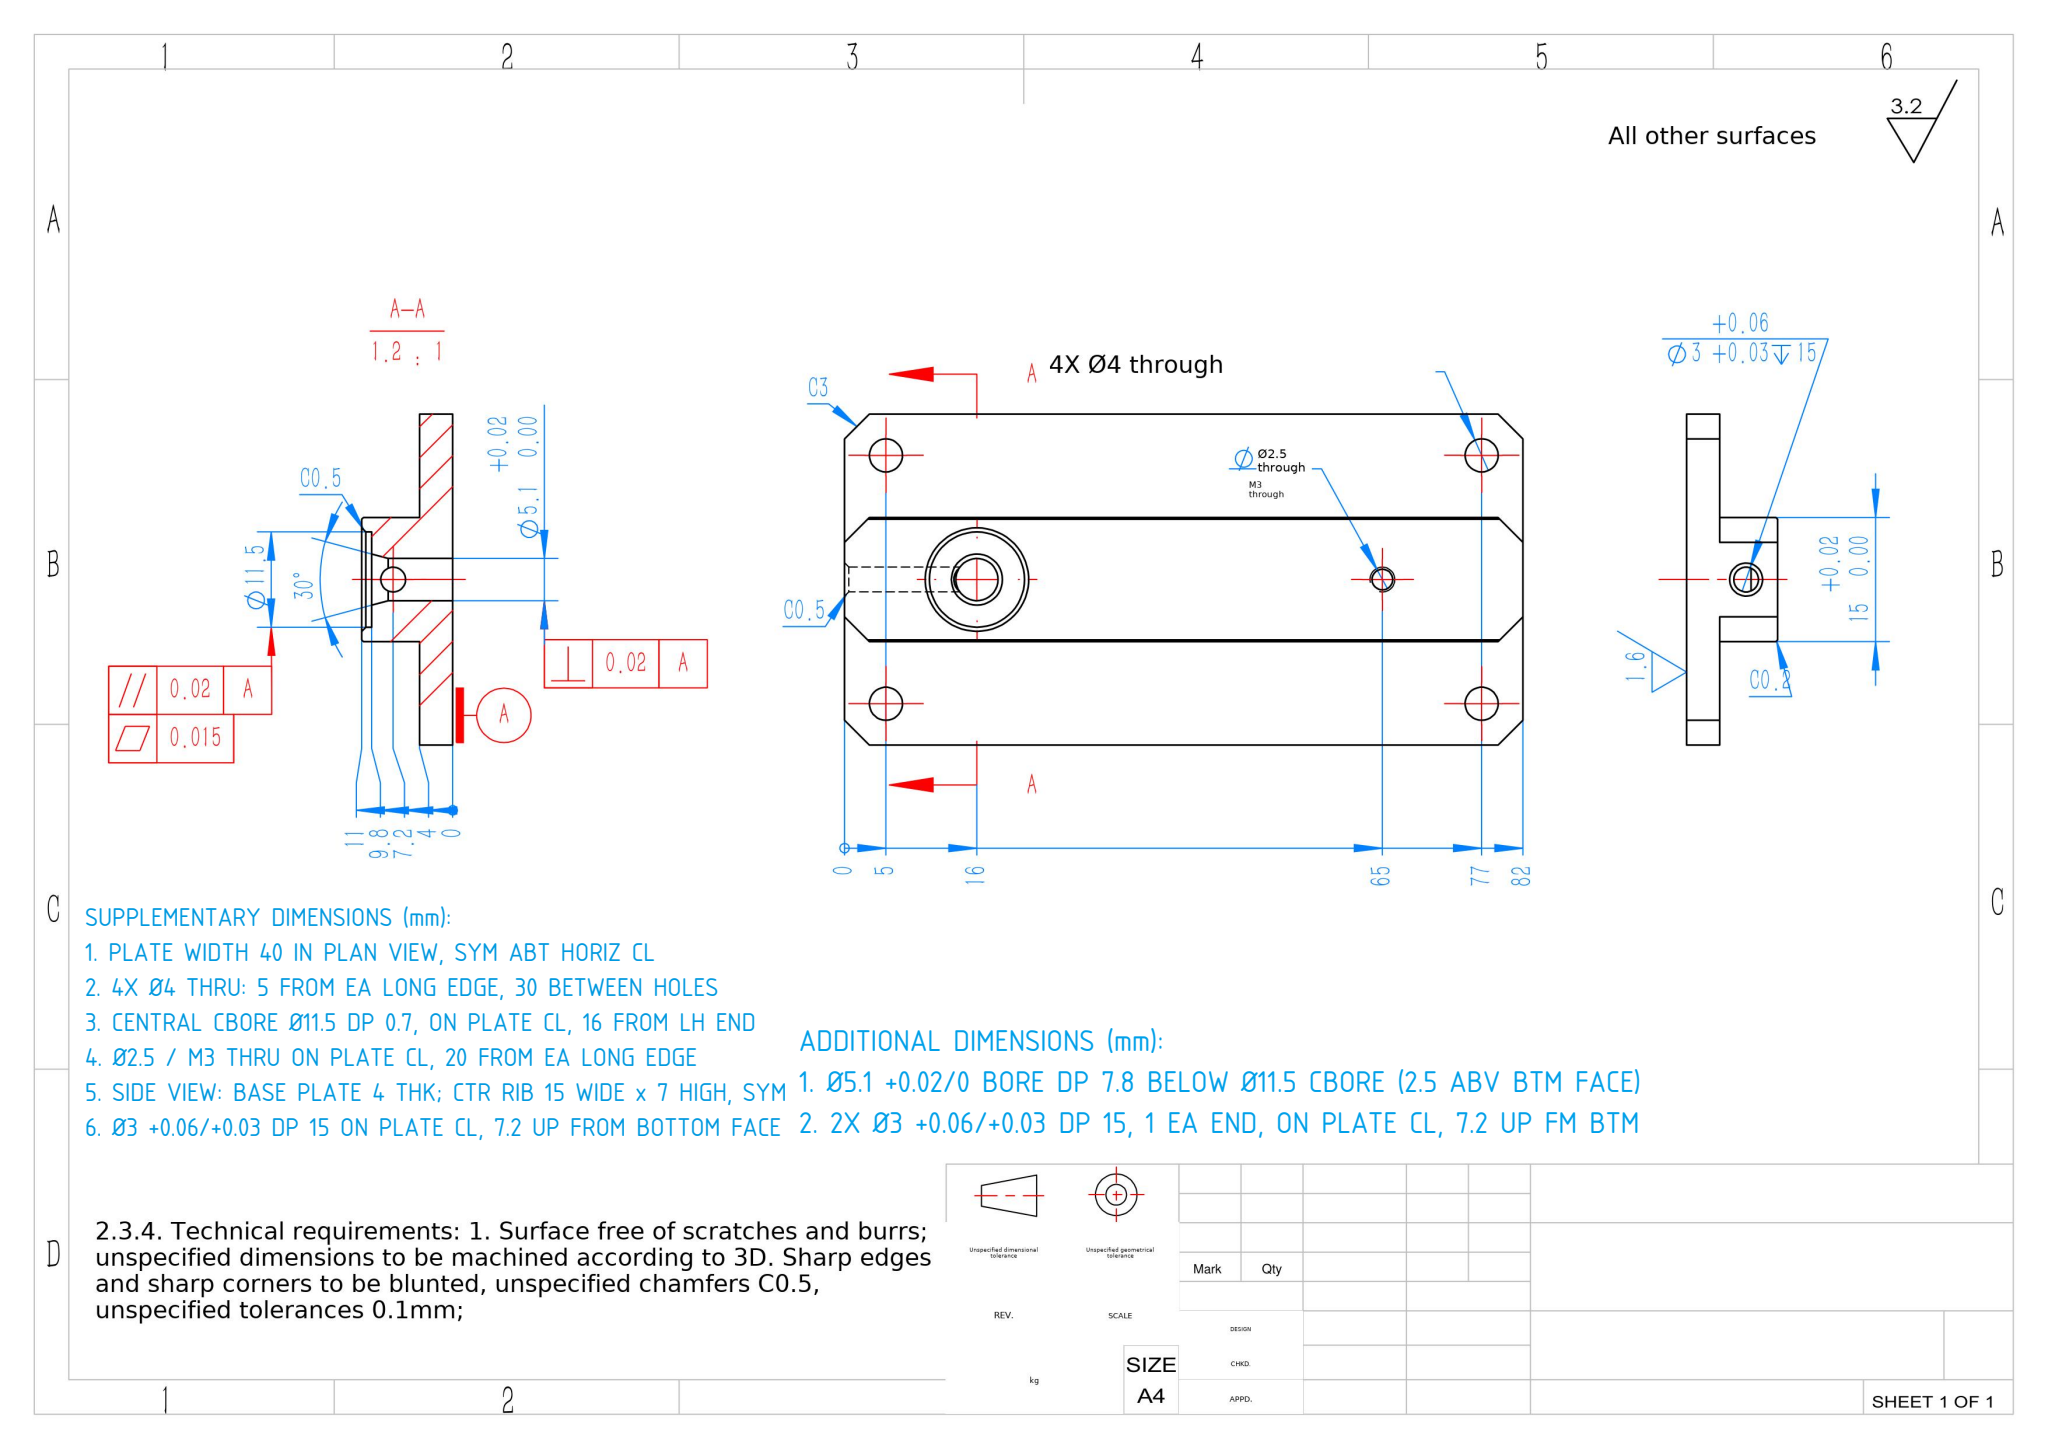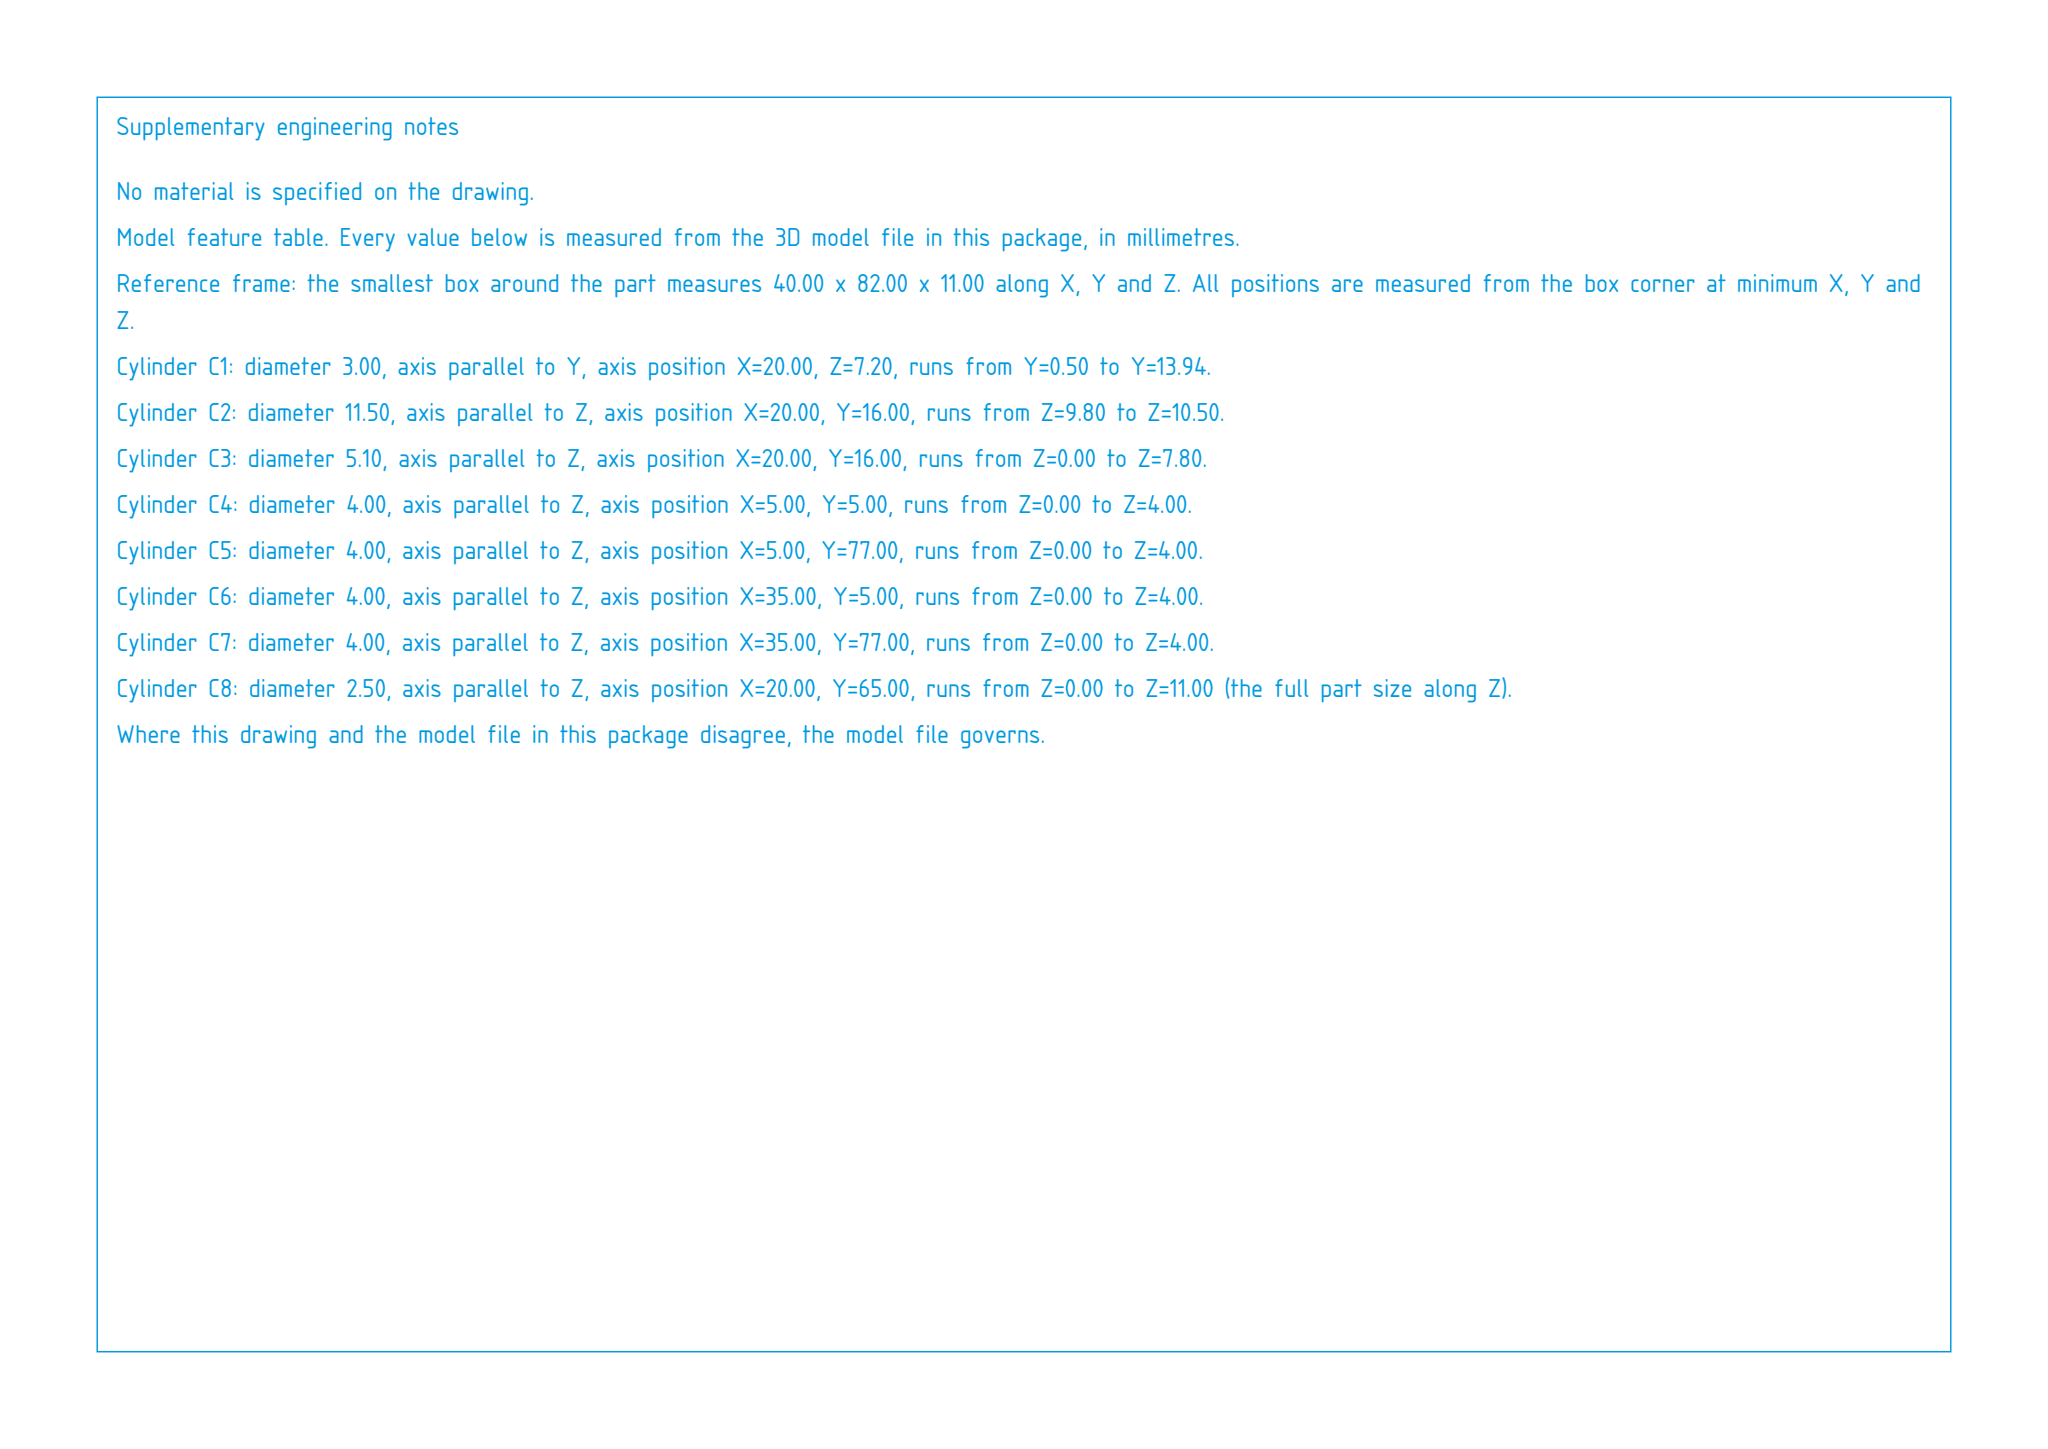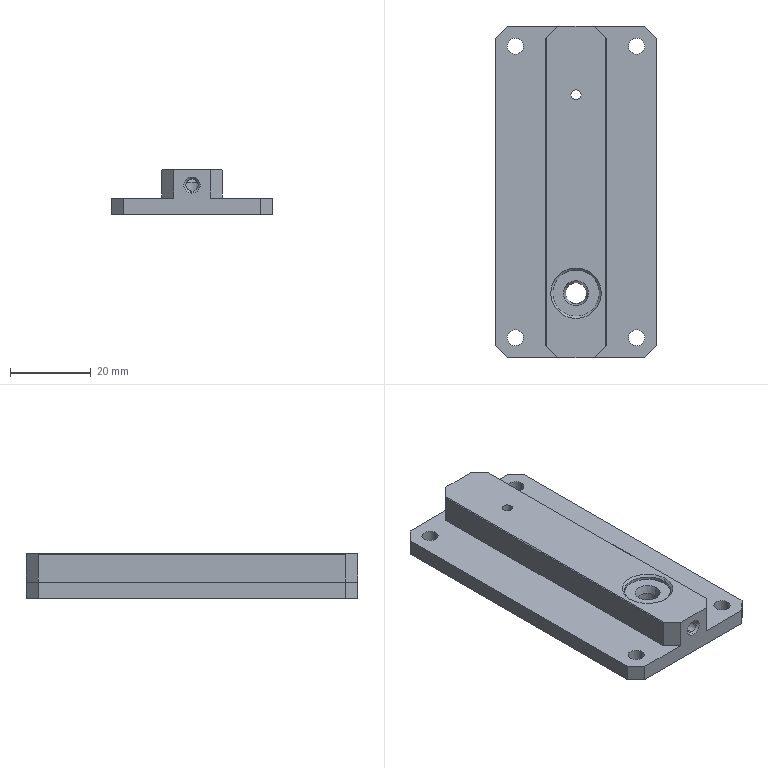Part | SolidWorks | mm | 1 solid | 43 faces | box 40 x 82 x 11 mm | volume 20838 mm3 | plane 21 | cylinder 16 | cone 6 | commonest cylinder face diameters 4 x8 3 x2 2.5 x2 5.1 x2 11.5 x2
build123d program:
from build123d import *

# Parameters (mm, degrees)
SKETCH1_W                     = 15
SKETCH1_H                     = 82
BOSS_EXTRUDE1_DEPTH           = 11
SKETCH14_W                    = 40
SKETCH14_H                    = 82
BOSS_EXTRUDE3_DEPTH           = 4
SKETCH3_R                     = 5.75
CUT_EXTRUDE2_DEPTH            = 1.2
F_5_2_5_2_DIAMETER_HOLE1_D    = 5.1
CHAMFER1_SIZE                 = 0.5
CHAMFER2_SIZE                 = 2
CHAMFER2_SIZE2                = 0.5359
M3_TAPPED_HOLE1_D             = 2.5
SIZE_MM_DOWEL_PIN_HOLE1_D     = 3
SIZE_MM_DOWEL_PIN_HOLE1_DEPTH = 15
SIZE_MM_DOWEL_PIN_HOLE1_TIP   = 0.9013
CHAMFER3_SIZE                 = 0.5
F_4_0_4_DIAMETER_HOLE1_D      = 4
CHAMFER4_SIZE                 = 3
CHAMFER5_SIZE                 = 3
CHAMFER6_SIZE                 = 0.2


with BuildPart() as part:
    # Sketch1 → Boss-Extrude1 (new body)
    with BuildSketch(Plane.XY):
        Rectangle(SKETCH1_W, SKETCH1_H)
    extrude(amount=BOSS_EXTRUDE1_DEPTH)

    # Sketch14 → Boss-Extrude3 (add)
    with BuildSketch(Plane(origin=(0, 0, 0), x_dir=(-1, 0, 0), z_dir=(0, 0, -1))):
        Rectangle(SKETCH14_W, SKETCH14_H)
    extrude(amount=-BOSS_EXTRUDE3_DEPTH)

    # Sketch3 → Cut-Extrude2 (cut)
    with BuildSketch(Plane.XY.offset(11)):
        with Locations((0, -25)):
            Circle(SKETCH3_R)
    extrude(amount=-CUT_EXTRUDE2_DEPTH, mode=Mode.SUBTRACT)

    # 5.2 _5.2_ Diameter Hole1 (through all)
    with Locations(Plane.XY.offset(9.8)):
        with Locations((0, -25)):
            Hole(F_5_2_5_2_DIAMETER_HOLE1_D / 2)

    # Chamfer1
    chamfer1_edges = [part.edges().sort_by_distance(p)[0] for p in [
        (-5.75, -25, 11),
    ]]
    chamfer(chamfer1_edges, length=CHAMFER1_SIZE)

    # Chamfer2
    chamfer2_edges = [part.edges().sort_by_distance(p)[0] for p in [
        (2.55, -25, 9.8),
    ]]
    chamfer2_side = [part.faces().sort_by_distance(p)[0] for p in [
        (2.55, -25, 4.9),
    ]]
    chamfer(chamfer2_edges, length=CHAMFER2_SIZE, length2=CHAMFER2_SIZE2, reference=chamfer2_side[0])

    # M3 Tapped Hole1 (through all)
    with Locations(Plane(origin=(0, 0, 0), x_dir=(-1, 0, 0), z_dir=(0, 0, -1))):
        with Locations((0, 24)):
            Hole(M3_TAPPED_HOLE1_D / 2)

    # Size mm Dowel Pin Hole1
    with Locations(Plane(origin=(0, -41, 0), x_dir=(-1, 0, 0), z_dir=(0, -1, 0))):
        with Locations((0, -7.2)):
            Hole(SIZE_MM_DOWEL_PIN_HOLE1_D / 2, depth=SIZE_MM_DOWEL_PIN_HOLE1_DEPTH)
            with Locations((0, 0, -(SIZE_MM_DOWEL_PIN_HOLE1_DEPTH + SIZE_MM_DOWEL_PIN_HOLE1_TIP / 2))):  # 118° drill point
                Cone(0, SIZE_MM_DOWEL_PIN_HOLE1_D / 2, SIZE_MM_DOWEL_PIN_HOLE1_TIP, mode=Mode.SUBTRACT)

    # Chamfer3
    chamfer3_edges = [part.edges().sort_by_distance(p)[0] for p in [
        (-1.5, -41, 7.2),
    ]]
    chamfer(chamfer3_edges, length=CHAMFER3_SIZE)

    # 4.0 _4_ Diameter Hole1 (through all)
    with Locations(Plane.XY.offset(4)):
        with Locations((15, 36), (-15, 36), (-15, -36), (15, -36)):
            Hole(F_4_0_4_DIAMETER_HOLE1_D / 2)

    # Chamfer4
    chamfer4_edges = [part.edges().sort_by_distance(p)[0] for p in [
        (-20, -41, 2),
        (20, 41, 2),
        (-20, 41, 2),
        (20, -41, 2),
    ]]
    chamfer(chamfer4_edges, length=CHAMFER4_SIZE)

    # Chamfer5
    chamfer5_edges = [part.edges().sort_by_distance(p)[0] for p in [
        (7.5, -41, 7.5),
        (-7.5, -41, 7.5),
        (-7.5, 41, 7.5),
        (7.5, 41, 7.5),
    ]]
    chamfer(chamfer5_edges, length=CHAMFER5_SIZE)

    # Chamfer6
    chamfer6_edges = [part.edges().sort_by_distance(p)[0] for p in [
        (-7.5, 0, 11),
        (7.5, 0, 11),
    ]]
    chamfer(chamfer6_edges, length=CHAMFER6_SIZE)


solid = part.part